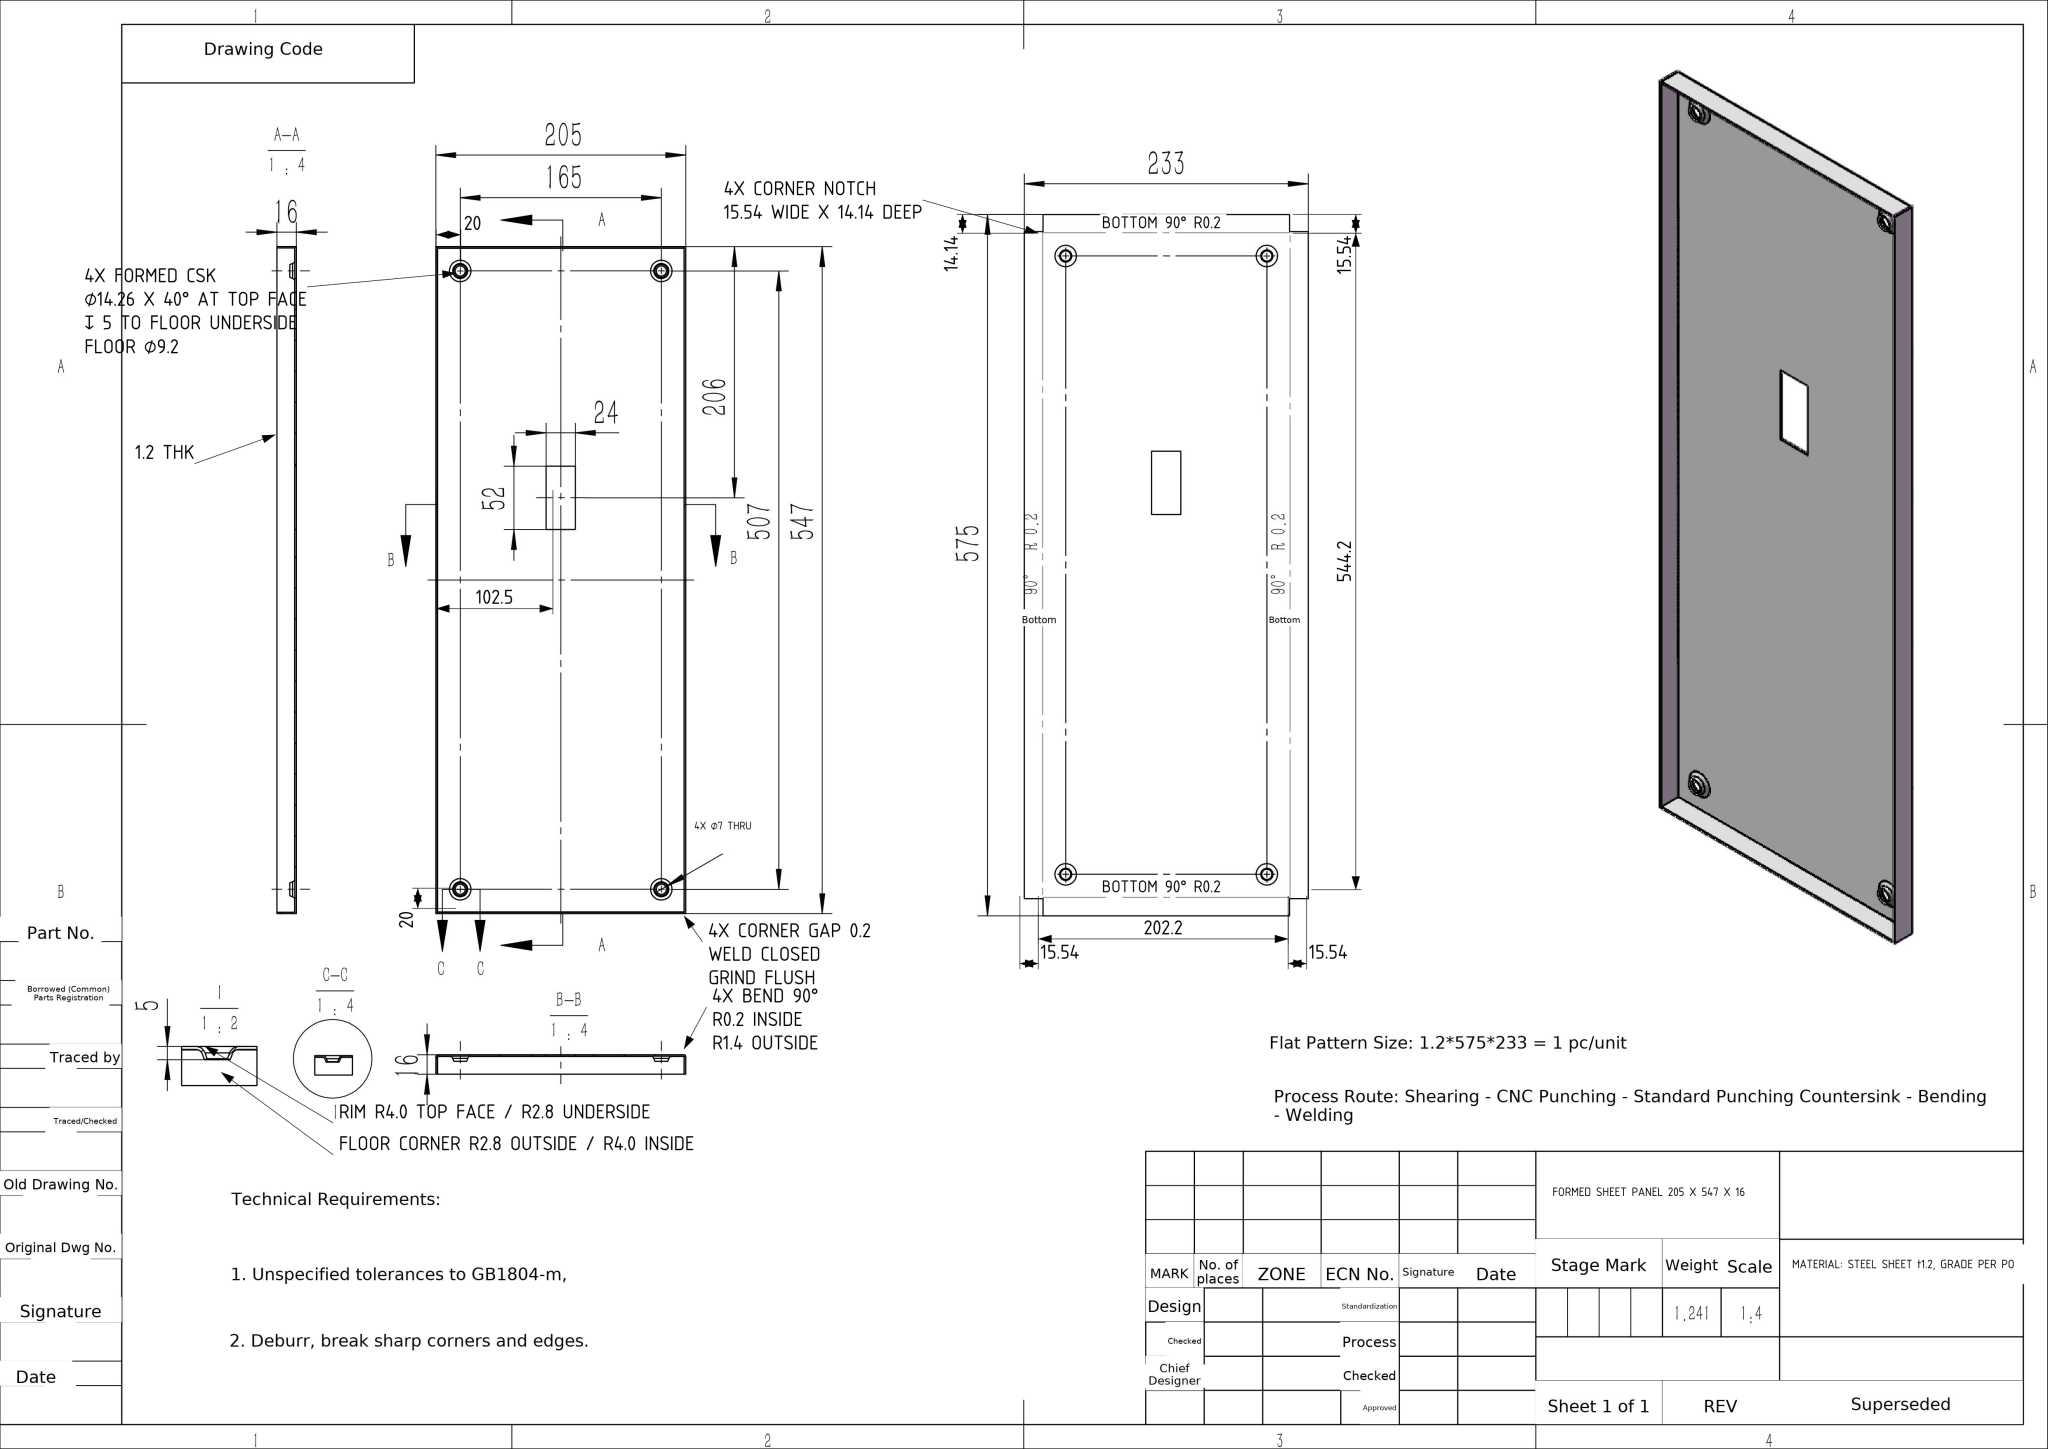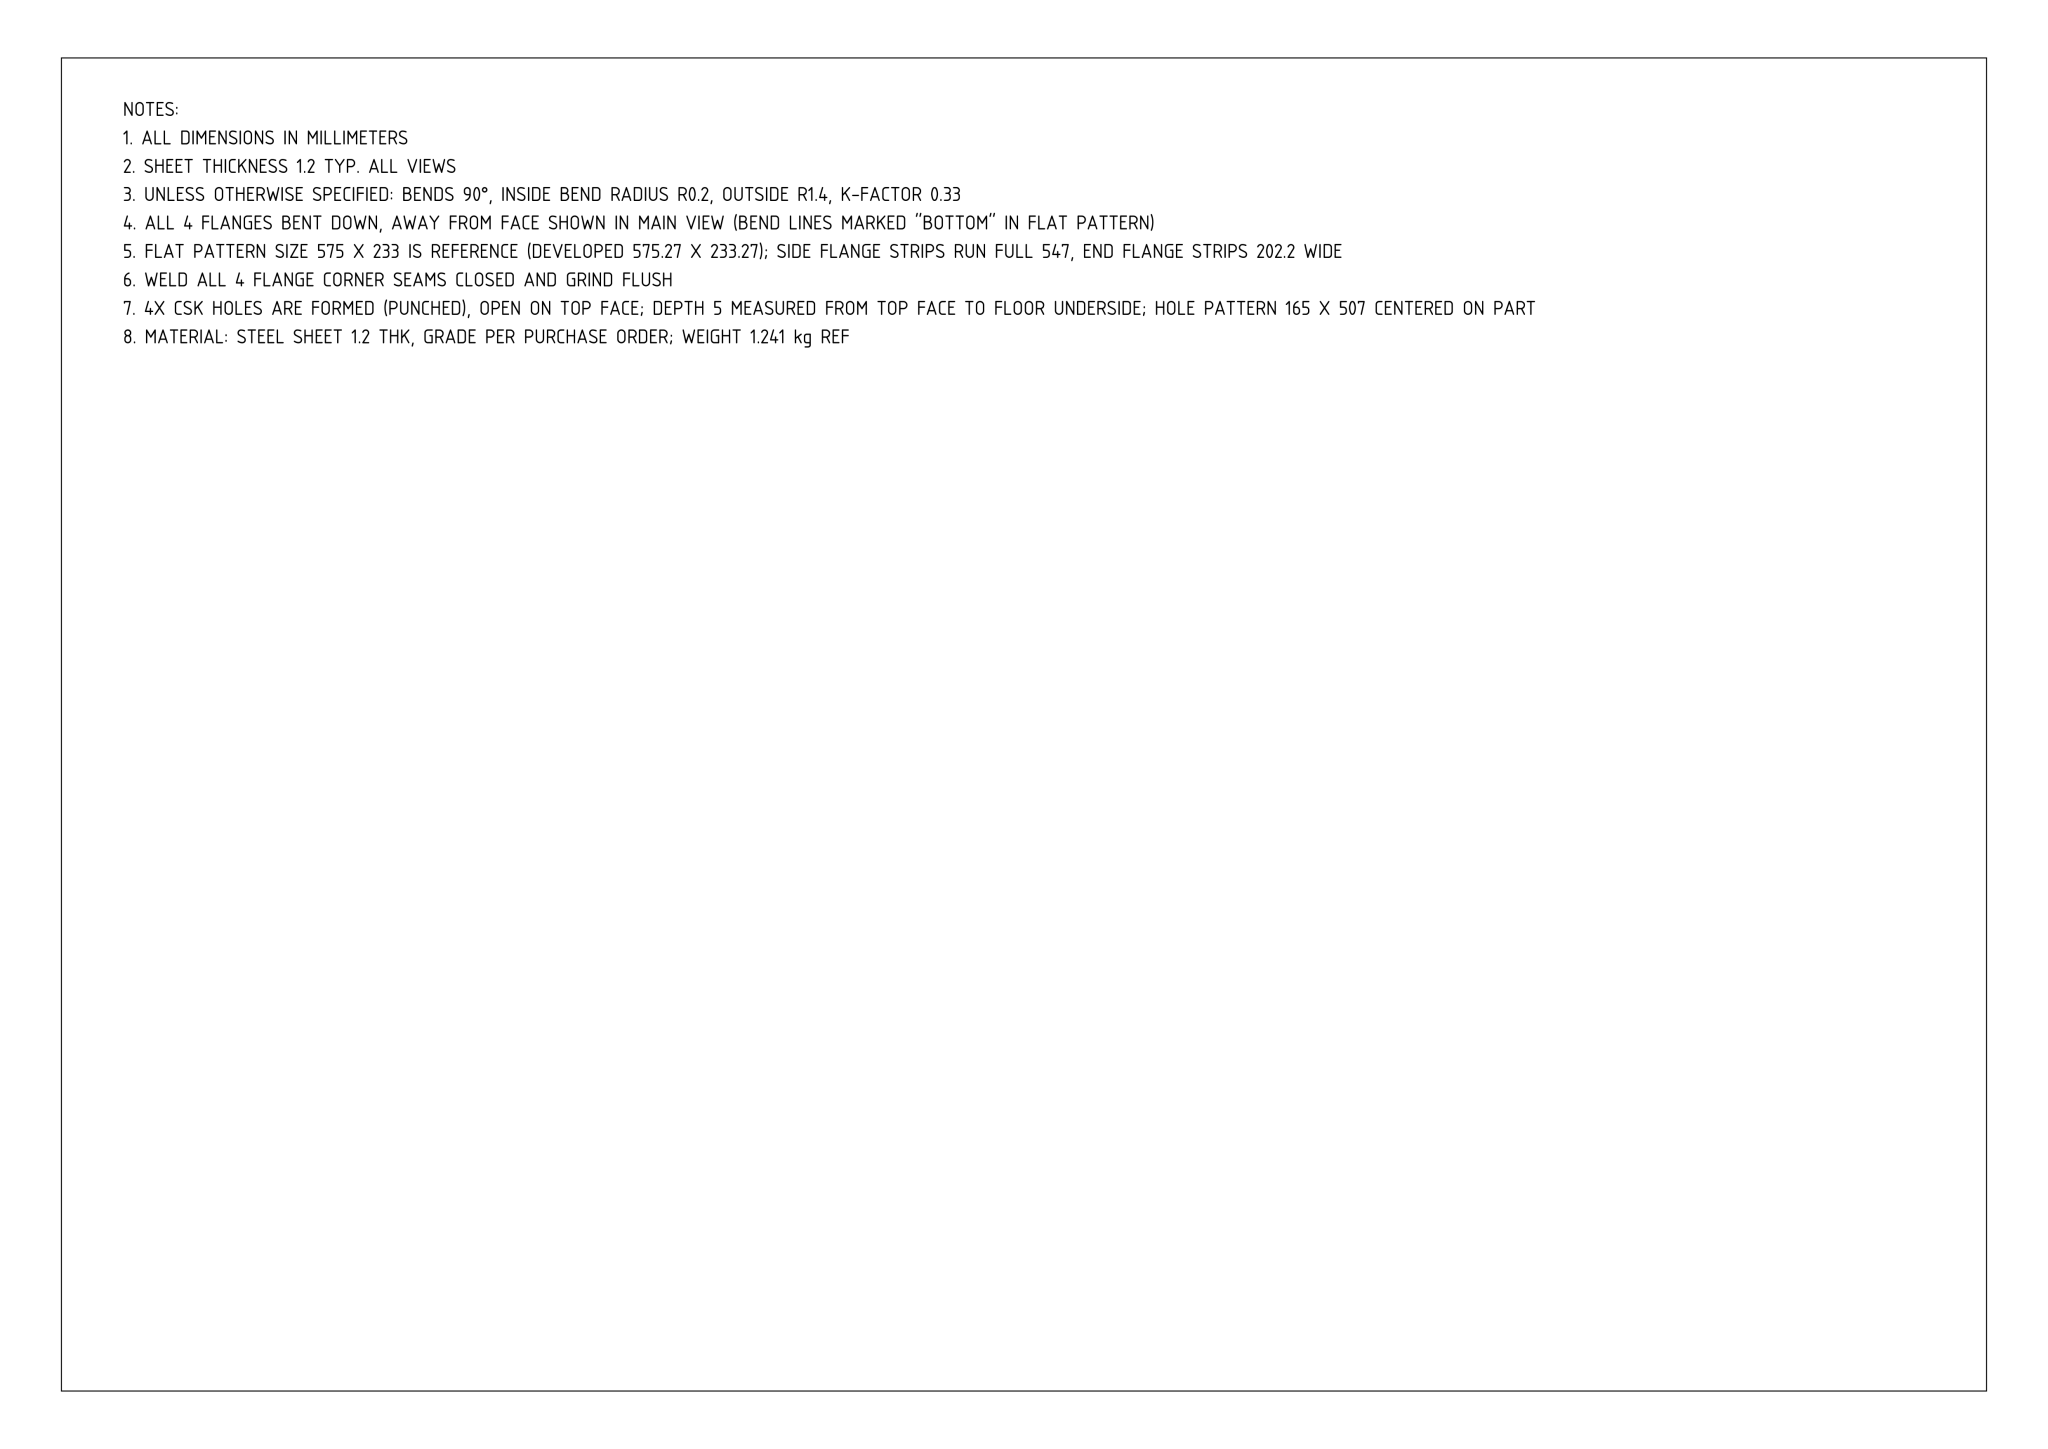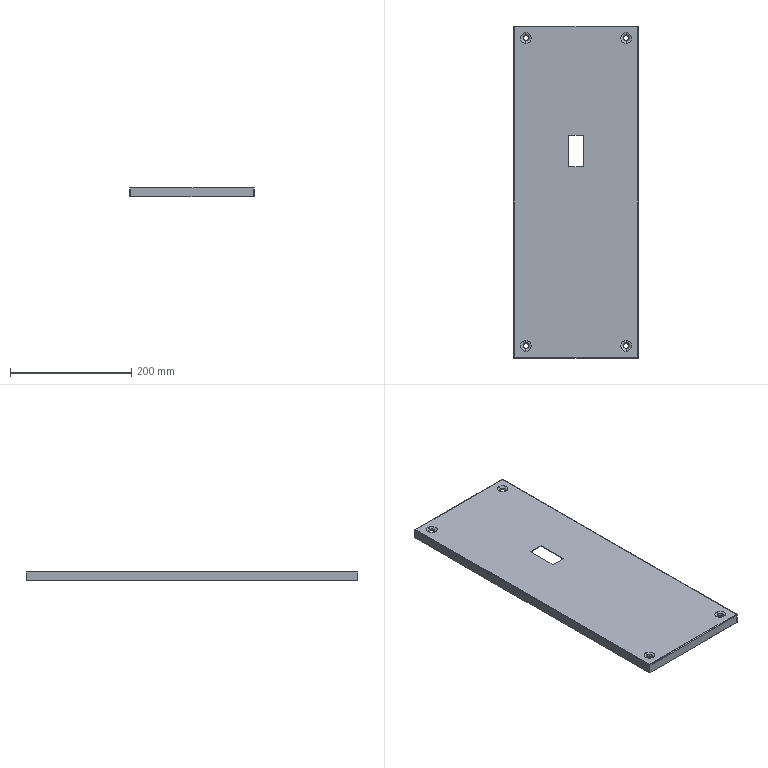Part | NX | mm | 1 solid | 86 faces | box 205 x 547 x 16 mm | volume 159155 mm3 | plane 38 | cone 24 | torus 16 | cylinder 8 | commonest cylinder face diameters 2.8 x4 0.4 x4